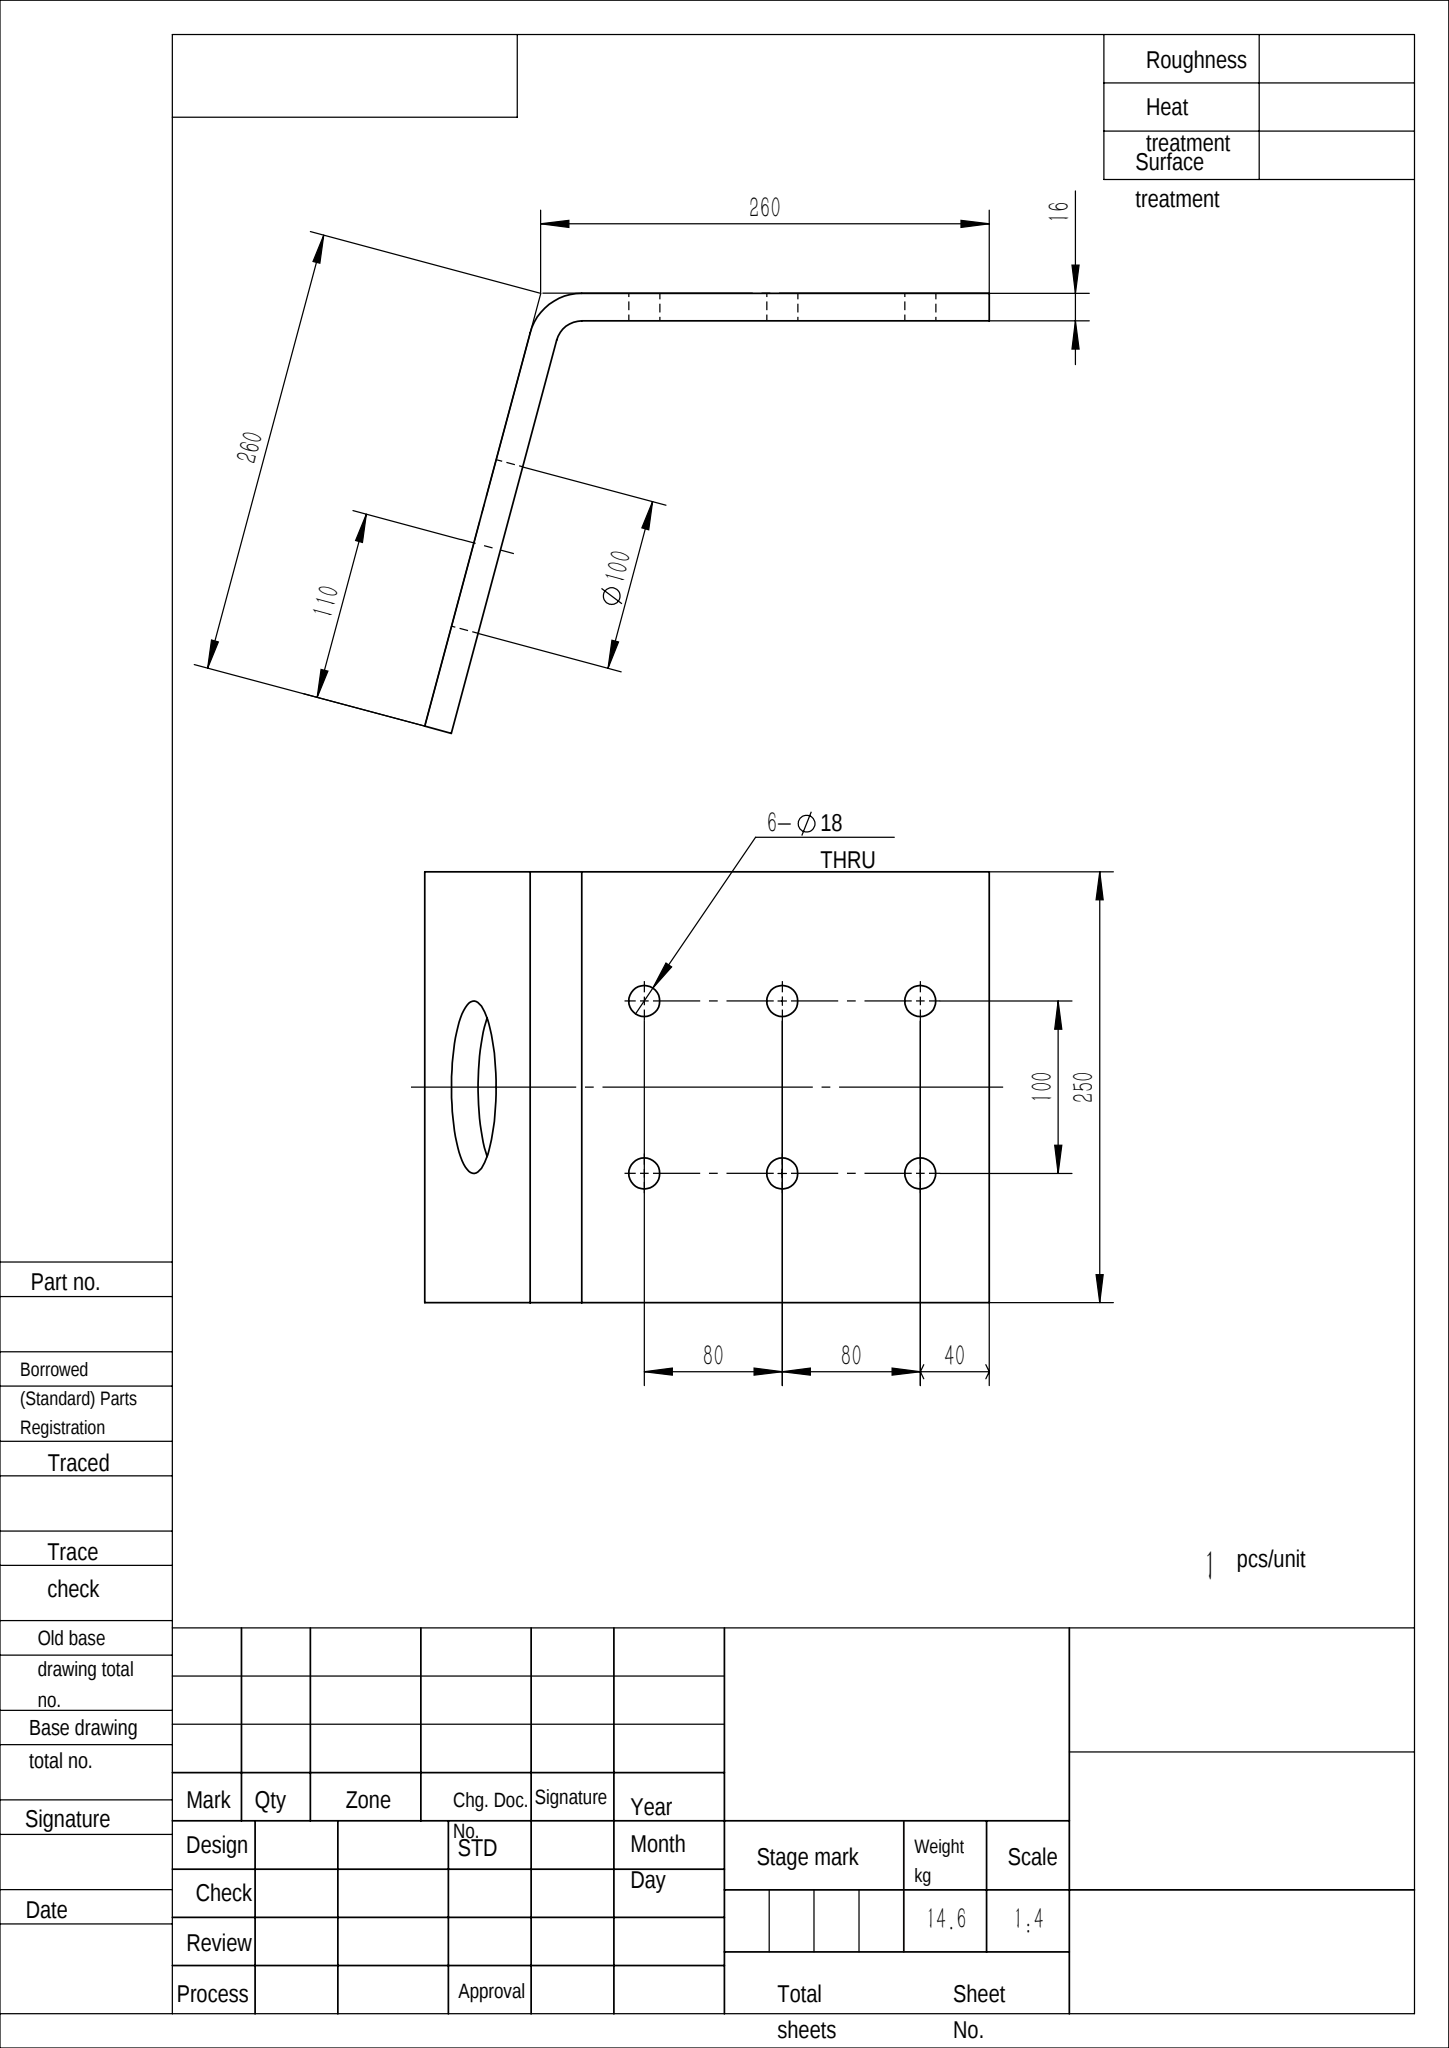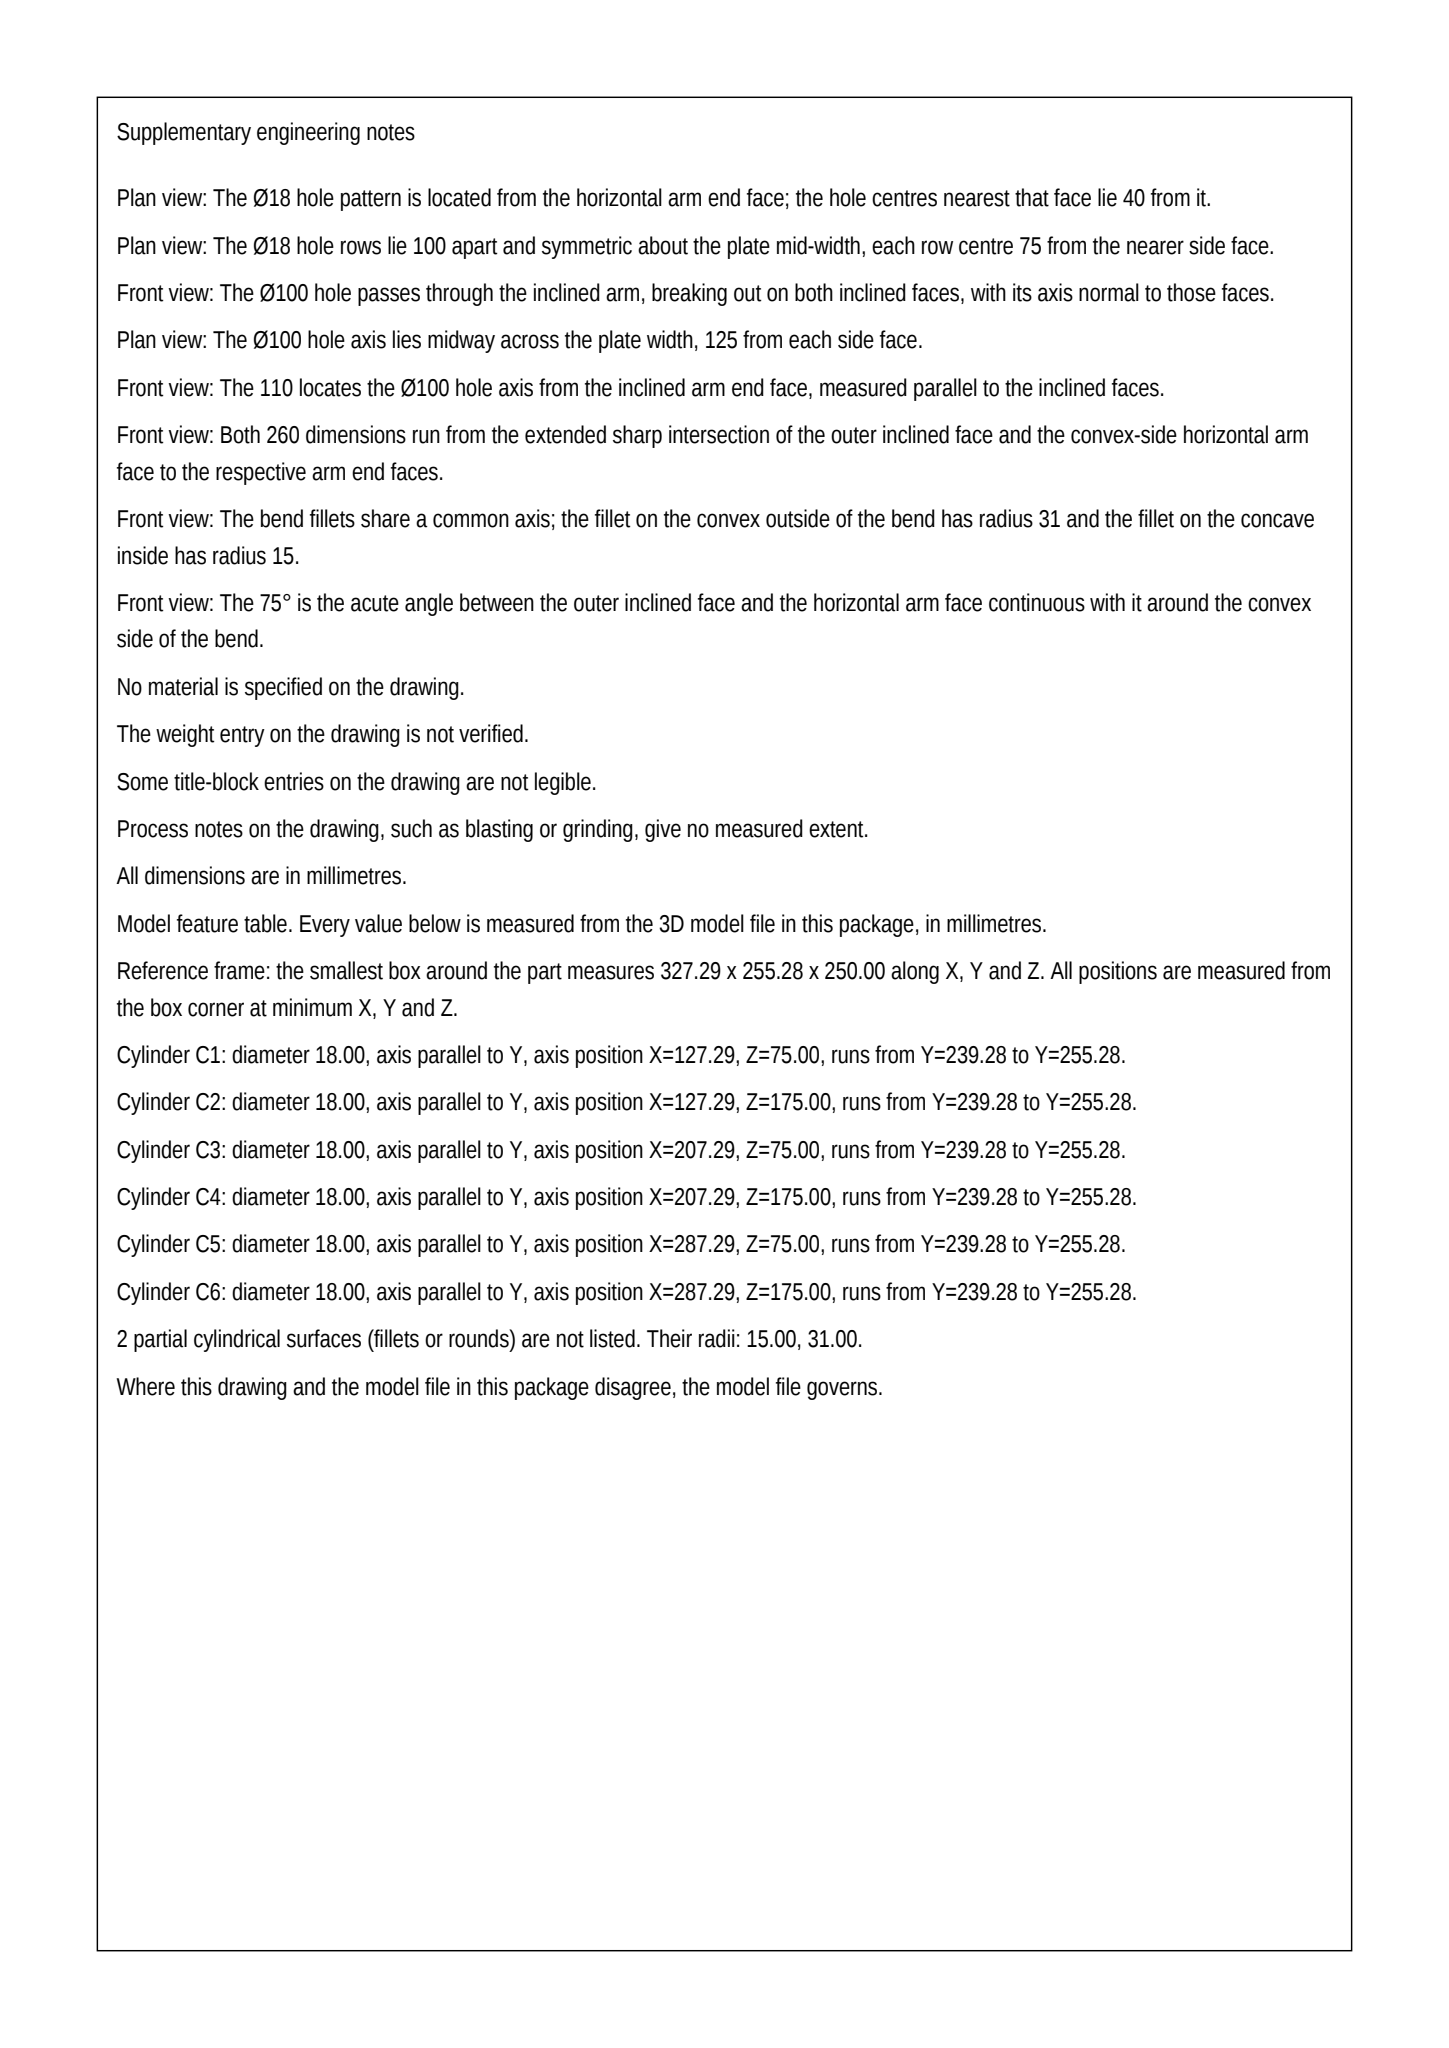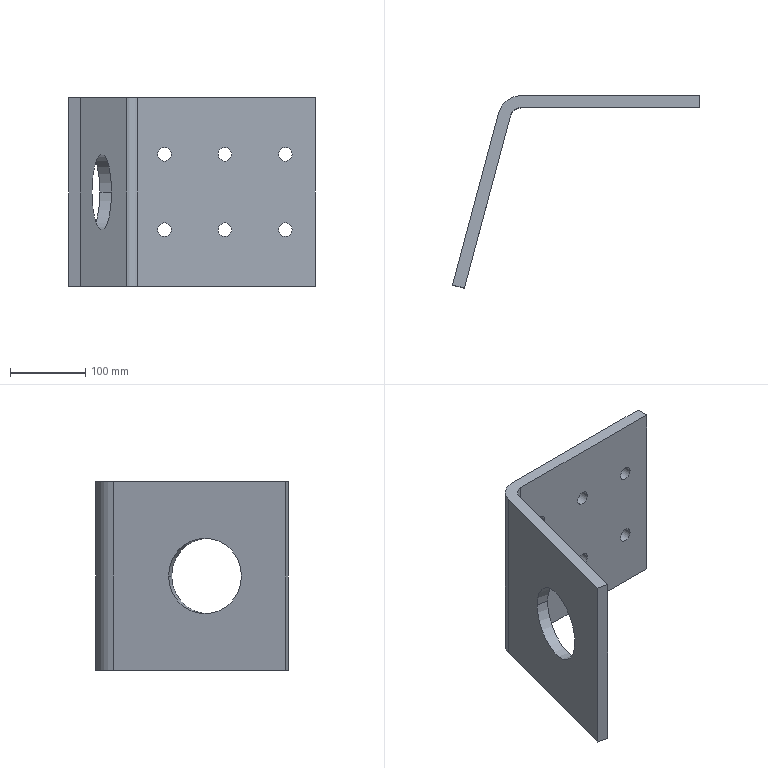Part | SolidWorks | mm | 1 solid | 24 faces | box 327.29 x 255.28 x 250 mm | volume 1860038 mm3 | cylinder 16 | plane 8 | commonest cylinder face diameters 18 x12 100 x2 30 x1 62 x1
Drawing notes:
INCLINED ARM THK 16 (UNIFORM W/ HORIZ ARM) | from the solid: Parallel faces y=239.28 & y=255.28 give 16 wall; holes len 16
① BEND ANGLE 105° BETWEEN FLAT ARM & INCLINED ARM | from the solid: Bent plate, t=16 (y 239.28 to 255.28), 250 wide (z 0 to 250); inclined arm meets horizontal arm at 105° included angle per model geometry
② R15 INSIDE BEND RAD AT 105° BEND | from the solid: Bend transition on 16 thk plate; inner bend face radius 15 (outer = 31)
build123d program:
from build123d import *

# Parameters (mm, degrees)
BOSS_EXTRUDE1_DEPTH = 125
CUT_EXTRUDE1_REACH  = 387.219
SKETCH2_R           = 9
LPATTERN1_COUNT     = 3
LPATTERN1_PITCH     = 80
SKETCH3_R           = 50
CUT_EXTRUDE2_DEPTH  = 373.155


with BuildPart() as part:
    # Sketch1 → Boss-Extrude1 (new, symmetric)
    with BuildSketch(Plane.XY):
        with BuildLine():
            Line((-67.293, -251.141), (-6.157, -22.977))
            ThreePointArc((-6.157, -22.977), (4.916, -6.406), (23.787, 0))
            Line((23.787, 0), (260, 0))
            Line((260, 0), (260, -16))
            Line((260, -16), (23.787, -16))
            ThreePointArc((23.787, -16), (14.656, -19.1), (9.298, -27.118))
            Line((9.298, -27.118), (-51.838, -255.282))
            Line((-51.838, -255.282), (-67.293, -251.141))
        make_face()
    extrude(amount=BOSS_EXTRUDE1_DEPTH, both=True)

    # Sketch2 → Cut-Extrude1 (cut, up to next)
    with BuildSketch(Plane(origin=(0, 0, 0), x_dir=(1, 0, 0), z_dir=(0, 1, 0)), mode=Mode.PRIVATE) as cut_extrude1_sk1:
        with Locations(Location((220, 50, 0), (0, 0, 180))):
            Circle(SKETCH2_R)
    cut_extrude1_tool1 = extrude(cut_extrude1_sk1.sketch, amount=-CUT_EXTRUDE1_REACH, mode=Mode.PRIVATE) & part.part
    # Sketch2 → Cut-Extrude1 (cut, up to next)
    with BuildSketch(Plane(origin=(0, 0, 0), x_dir=(1, 0, 0), z_dir=(0, 1, 0)), mode=Mode.PRIVATE) as cut_extrude1_sk2:
        with Locations(Location((220, -50, 0), (0, 0, 180))):
            Circle(SKETCH2_R)
    cut_extrude1_tool2 = extrude(cut_extrude1_sk2.sketch, amount=-CUT_EXTRUDE1_REACH, mode=Mode.PRIVATE) & part.part
    cut_extrude1_1 = cut_extrude1_tool1.solids().sort_by_distance((220, 0, -50))[0]
    add(cut_extrude1_1, mode=Mode.SUBTRACT)
    cut_extrude1_2 = cut_extrude1_tool2.solids().sort_by_distance((220, 0, 50))[0]
    add(cut_extrude1_2, mode=Mode.SUBTRACT)
    cut_extrude1 = cut_extrude1_1 + cut_extrude1_2  # Cut-Extrude1 as one shape, for the pattern or mirror that repeats it

    # LPattern1: Cut-Extrude1 ×3
    with Locations(*[(-i * LPATTERN1_PITCH, 0, 0) for i in range(1, LPATTERN1_COUNT)]):
        add(cut_extrude1, mode=Mode.SUBTRACT)

    # Sketch3 → Cut-Extrude2 (cut, through all)
    with BuildSketch(Plane(origin=(15.455, -4.141, 0), x_dir=(0, 0, -1), z_dir=(0.9659, -0.2588, 0))):
        with Locations(Location((0, -150, 0), (0, 0, 90))):
            Circle(SKETCH3_R)
    extrude(amount=-CUT_EXTRUDE2_DEPTH, mode=Mode.SUBTRACT)


solid = part.part
STEP:
#1=CARTESIAN_POINT('',(-51.764,-193.185,0.));
#2=VERTEX_POINT('',#1);
#3=CARTESIAN_POINT('',(-25.882,-96.593,-0.));
#4=VERTEX_POINT('',#3);
#5=CARTESIAN_POINT('',(-38.823,-144.889,0.));
#6=DIRECTION('',(0.9659,-0.2588,-0.));
#7=DIRECTION('',(0.2588,0.9659,0.));
#8=AXIS2_PLACEMENT_3D('',#5,#6,#7);
#9=CIRCLE('',#8,50.);
#10=EDGE_CURVE('',#2,#4,#9,.T.);
#11=ORIENTED_EDGE('',*,*,#10,.F.);
#12=CARTESIAN_POINT('',(-36.309,-197.326,0.));
#13=VERTEX_POINT('',#12);
#14=CARTESIAN_POINT('',(-114.549,-176.362,0.));
#15=DIRECTION('',(0.9659,-0.2588,-0.));
#16=VECTOR('',#15,1000.);
#17=LINE('',#14,#16);
#18=EDGE_CURVE('',#2,#13,#17,.T.);
#19=ORIENTED_EDGE('',*,*,#18,.T.);
#20=CARTESIAN_POINT('',(-10.427,-100.734,-0.));
#21=VERTEX_POINT('',#20);
#22=CARTESIAN_POINT('',(-23.368,-149.03,-0.));
#23=DIRECTION('',(0.9659,-0.2588,-0.));
#24=DIRECTION('',(0.2588,0.9659,0.));
#25=AXIS2_PLACEMENT_3D('',#22,#23,#24);
#26=CIRCLE('',#25,50.);
#27=EDGE_CURVE('',#13,#21,#26,.T.);
#28=ORIENTED_EDGE('',*,*,#27,.T.);
#29=CARTESIAN_POINT('',(-88.667,-79.769,0.));
#30=DIRECTION('',(0.9659,-0.2588,-0.));
#31=VECTOR('',#30,1000.);
#32=LINE('',#29,#31);
#33=EDGE_CURVE('',#4,#21,#32,.T.);
#34=ORIENTED_EDGE('',*,*,#33,.F.);
#35=EDGE_LOOP('',(#11,#19,#28,#34));
#36=FACE_OUTER_BOUND('',#35,.T.);
#37=CARTESIAN_POINT('',(-101.608,-128.066,0.));
#38=DIRECTION('',(0.9659,-0.2588,-0.));
#39=DIRECTION('',(0.2588,0.9659,0.));
#40=AXIS2_PLACEMENT_3D('',#37,#38,#39);
#41=CYLINDRICAL_SURFACE('',#40,50.);
#42=ADVANCED_FACE('',(#36),#41,.F.);
#43=CARTESIAN_POINT('',(131.,-16.,-50.));
#44=VERTEX_POINT('',#43);
#45=CARTESIAN_POINT('',(149.,-16.,-50.));
#46=VERTEX_POINT('',#45);
#47=CARTESIAN_POINT('',(140.,-16.,-50.));
#48=DIRECTION('',(0.,-1.,-0.));
#49=DIRECTION('',(-1.,-0.,0.));
#50=AXIS2_PLACEMENT_3D('',#47,#48,#49);
#51=CIRCLE('',#50,9.);
#52=EDGE_CURVE('',#44,#46,#51,.T.);
#53=ORIENTED_EDGE('',*,*,#52,.T.);
#54=CARTESIAN_POINT('',(149.,-0.,-50.));
#55=VERTEX_POINT('',#54);
#56=CARTESIAN_POINT('',(149.,-255.283,-50.));
#57=DIRECTION('',(-0.,1.,0.));
#58=VECTOR('',#57,1000.);
#59=LINE('',#56,#58);
#60=EDGE_CURVE('',#46,#55,#59,.T.);
#61=ORIENTED_EDGE('',*,*,#60,.T.);
#62=CARTESIAN_POINT('',(131.,-0.,-50.));
#63=VERTEX_POINT('',#62);
#64=CARTESIAN_POINT('',(140.,-0.,-50.));
#65=DIRECTION('',(-0.,1.,0.));
#66=DIRECTION('',(-1.,-0.,0.));
#67=AXIS2_PLACEMENT_3D('',#64,#65,#66);
#68=CIRCLE('',#67,9.);
#69=EDGE_CURVE('',#55,#63,#68,.T.);
#70=ORIENTED_EDGE('',*,*,#69,.T.);
#71=CARTESIAN_POINT('',(131.,-255.283,-50.));
#72=DIRECTION('',(-0.,1.,0.));
#73=VECTOR('',#72,1000.);
#74=LINE('',#71,#73);
#75=EDGE_CURVE('',#44,#63,#74,.T.);
#76=ORIENTED_EDGE('',*,*,#75,.F.);
#77=EDGE_LOOP('',(#53,#61,#70,#76));
#78=FACE_OUTER_BOUND('',#77,.T.);
#79=CARTESIAN_POINT('',(140.,-255.283,-50.));
#80=DIRECTION('',(-0.,1.,0.));
#81=DIRECTION('',(-1.,0.,0.));
#82=AXIS2_PLACEMENT_3D('',#79,#80,#81);
#83=CYLINDRICAL_SURFACE('',#82,9.);
#84=ADVANCED_FACE('',(#78),#83,.F.);
#85=CARTESIAN_POINT('',(131.,-16.,50.));
#86=VERTEX_POINT('',#85);
#87=CARTESIAN_POINT('',(149.,-16.,50.));
#88=VERTEX_POINT('',#87);
#89=CARTESIAN_POINT('',(140.,-16.,50.));
#90=DIRECTION('',(0.,-1.,-0.));
#91=DIRECTION('',(-1.,-0.,0.));
#92=AXIS2_PLACEMENT_3D('',#89,#90,#91);
#93=CIRCLE('',#92,9.);
#94=EDGE_CURVE('',#86,#88,#93,.T.);
#95=ORIENTED_EDGE('',*,*,#94,.T.);
#96=CARTESIAN_POINT('',(149.,-0.,50.));
#97=VERTEX_POINT('',#96);
#98=CARTESIAN_POINT('',(149.,-255.283,50.));
#99=DIRECTION('',(-0.,1.,0.));
#100=VECTOR('',#99,1000.);
#101=LINE('',#98,#100);
#102=EDGE_CURVE('',#88,#97,#101,.T.);
#103=ORIENTED_EDGE('',*,*,#102,.T.);
#104=CARTESIAN_POINT('',(131.,-0.,50.));
#105=VERTEX_POINT('',#104);
#106=CARTESIAN_POINT('',(140.,-0.,50.));
#107=DIRECTION('',(-0.,1.,0.));
#108=DIRECTION('',(-1.,-0.,0.));
#109=AXIS2_PLACEMENT_3D('',#106,#107,#108);
#110=CIRCLE('',#109,9.);
#111=EDGE_CURVE('',#97,#105,#110,.T.);
#112=ORIENTED_EDGE('',*,*,#111,.T.);
#113=CARTESIAN_POINT('',(131.,-255.283,50.));
#114=DIRECTION('',(-0.,1.,0.));
#115=VECTOR('',#114,1000.);
#116=LINE('',#113,#115);
#117=EDGE_CURVE('',#86,#105,#116,.T.);
#118=ORIENTED_EDGE('',*,*,#117,.F.);
#119=EDGE_LOOP('',(#95,#103,#112,#118));
#120=FACE_OUTER_BOUND('',#119,.T.);
#121=CARTESIAN_POINT('',(140.,-255.283,50.));
#122=DIRECTION('',(-0.,1.,0.));
#123=DIRECTION('',(-1.,0.,0.));
#124=AXIS2_PLACEMENT_3D('',#121,#122,#123);
#125=CYLINDRICAL_SURFACE('',#124,9.);
#126=ADVANCED_FACE('',(#120),#125,.F.);
#127=CARTESIAN_POINT('',(211.,-16.,50.));
#128=VERTEX_POINT('',#127);
#129=CARTESIAN_POINT('',(229.,-16.,50.));
#130=VERTEX_POINT('',#129);
#131=CARTESIAN_POINT('',(220.,-16.,50.));
#132=DIRECTION('',(0.,-1.,-0.));
#133=DIRECTION('',(-1.,-0.,0.));
#134=AXIS2_PLACEMENT_3D('',#131,#132,#133);
#135=CIRCLE('',#134,9.);
#136=EDGE_CURVE('',#128,#130,#135,.T.);
#137=ORIENTED_EDGE('',*,*,#136,.T.);
#138=CARTESIAN_POINT('',(229.,0.,50.));
#139=VERTEX_POINT('',#138);
#140=CARTESIAN_POINT('',(229.,-255.283,50.));
#141=DIRECTION('',(-0.,1.,0.));
#142=VECTOR('',#141,1000.);
#143=LINE('',#140,#142);
#144=EDGE_CURVE('',#130,#139,#143,.T.);
#145=ORIENTED_EDGE('',*,*,#144,.T.);
#146=CARTESIAN_POINT('',(211.,-0.,50.));
#147=VERTEX_POINT('',#146);
#148=CARTESIAN_POINT('',(220.,0.,50.));
#149=DIRECTION('',(-0.,1.,0.));
#150=DIRECTION('',(-1.,-0.,0.));
#151=AXIS2_PLACEMENT_3D('',#148,#149,#150);
#152=CIRCLE('',#151,9.);
#153=EDGE_CURVE('',#139,#147,#152,.T.);
#154=ORIENTED_EDGE('',*,*,#153,.T.);
#155=CARTESIAN_POINT('',(211.,-255.283,50.));
#156=DIRECTION('',(-0.,1.,0.));
#157=VECTOR('',#156,1000.);
#158=LINE('',#155,#157);
#159=EDGE_CURVE('',#128,#147,#158,.T.);
#160=ORIENTED_EDGE('',*,*,#159,.F.);
#161=EDGE_LOOP('',(#137,#145,#154,#160));
#162=FACE_OUTER_BOUND('',#161,.T.);
#163=CARTESIAN_POINT('',(220.,-255.283,50.));
#164=DIRECTION('',(-0.,1.,0.));
#165=DIRECTION('',(-1.,0.,0.));
#166=AXIS2_PLACEMENT_3D('',#163,#164,#165);
#167=CYLINDRICAL_SURFACE('',#166,9.);
#168=ADVANCED_FACE('',(#162),#167,.F.);
#169=CARTESIAN_POINT('',(211.,-16.,-50.));
#170=VERTEX_POINT('',#169);
#171=CARTESIAN_POINT('',(229.,-16.,-50.));
#172=VERTEX_POINT('',#171);
#173=CARTESIAN_POINT('',(220.,-16.,-50.));
#174=DIRECTION('',(0.,-1.,-0.));
#175=DIRECTION('',(-1.,-0.,0.));
#176=AXIS2_PLACEMENT_3D('',#173,#174,#175);
#177=CIRCLE('',#176,9.);
#178=EDGE_CURVE('',#170,#172,#177,.T.);
#179=ORIENTED_EDGE('',*,*,#178,.T.);
#180=CARTESIAN_POINT('',(229.,0.,-50.));
#181=VERTEX_POINT('',#180);
#182=CARTESIAN_POINT('',(229.,-255.283,-50.));
#183=DIRECTION('',(-0.,1.,0.));
#184=VECTOR('',#183,1000.);
#185=LINE('',#182,#184);
#186=EDGE_CURVE('',#172,#181,#185,.T.);
#187=ORIENTED_EDGE('',*,*,#186,.T.);
#188=CARTESIAN_POINT('',(211.,-0.,-50.));
#189=VERTEX_POINT('',#188);
#190=CARTESIAN_POINT('',(220.,0.,-50.));
#191=DIRECTION('',(-0.,1.,0.));
#192=DIRECTION('',(-1.,-0.,0.));
#193=AXIS2_PLACEMENT_3D('',#190,#191,#192);
#194=CIRCLE('',#193,9.);
#195=EDGE_CURVE('',#181,#189,#194,.T.);
#196=ORIENTED_EDGE('',*,*,#195,.T.);
#197=CARTESIAN_POINT('',(211.,-255.283,-50.));
#198=DIRECTION('',(-0.,1.,0.));
#199=VECTOR('',#198,1000.);
#200=LINE('',#197,#199);
#201=EDGE_CURVE('',#170,#189,#200,.T.);
#202=ORIENTED_EDGE('',*,*,#201,.F.);
#203=EDGE_LOOP('',(#179,#187,#196,#202));
#204=FACE_OUTER_BOUND('',#203,.T.);
#205=CARTESIAN_POINT('',(220.,-255.283,-50.));
#206=DIRECTION('',(-0.,1.,0.));
#207=DIRECTION('',(-1.,0.,0.));
#208=AXIS2_PLACEMENT_3D('',#205,#206,#207);
#209=CYLINDRICAL_SURFACE('',#208,9.);
#210=ADVANCED_FACE('',(#204),#209,.F.);
#211=CARTESIAN_POINT('',(51.,-16.,50.));
#212=VERTEX_POINT('',#211);
#213=CARTESIAN_POINT('',(69.,-16.,50.));
#214=VERTEX_POINT('',#213);
#215=CARTESIAN_POINT('',(60.,-16.,50.));
#216=DIRECTION('',(0.,-1.,-0.));
#217=DIRECTION('',(-1.,-0.,0.));
#218=AXIS2_PLACEMENT_3D('',#215,#216,#217);
#219=CIRCLE('',#218,9.);
#220=EDGE_CURVE('',#212,#214,#219,.T.);
#221=ORIENTED_EDGE('',*,*,#220,.T.);
#222=CARTESIAN_POINT('',(69.,0.,50.));
#223=VERTEX_POINT('',#222);
#224=CARTESIAN_POINT('',(69.,-255.283,50.));
#225=DIRECTION('',(-0.,1.,0.));
#226=VECTOR('',#225,1000.);
#227=LINE('',#224,#226);
#228=EDGE_CURVE('',#214,#223,#227,.T.);
#229=ORIENTED_EDGE('',*,*,#228,.T.);
#230=CARTESIAN_POINT('',(51.,-0.,50.));
#231=VERTEX_POINT('',#230);
#232=CARTESIAN_POINT('',(60.,0.,50.));
#233=DIRECTION('',(-0.,1.,0.));
#234=DIRECTION('',(-1.,-0.,0.));
#235=AXIS2_PLACEMENT_3D('',#232,#233,#234);
#236=CIRCLE('',#235,9.);
#237=EDGE_CURVE('',#223,#231,#236,.T.);
#238=ORIENTED_EDGE('',*,*,#237,.T.);
#239=CARTESIAN_POINT('',(51.,-255.283,50.));
#240=DIRECTION('',(-0.,1.,0.));
#241=VECTOR('',#240,1000.);
#242=LINE('',#239,#241);
#243=EDGE_CURVE('',#212,#231,#242,.T.);
#244=ORIENTED_EDGE('',*,*,#243,.F.);
#245=EDGE_LOOP('',(#221,#229,#238,#244));
#246=FACE_OUTER_BOUND('',#245,.T.);
#247=CARTESIAN_POINT('',(60.,-255.283,50.));
#248=DIRECTION('',(-0.,1.,0.));
#249=DIRECTION('',(-1.,0.,0.));
#250=AXIS2_PLACEMENT_3D('',#247,#248,#249);
#251=CYLINDRICAL_SURFACE('',#250,9.);
#252=ADVANCED_FACE('',(#246),#251,.F.);
#253=CARTESIAN_POINT('',(51.,-16.,-50.));
#254=VERTEX_POINT('',#253);
#255=CARTESIAN_POINT('',(69.,-16.,-50.));
#256=VERTEX_POINT('',#255);
#257=CARTESIAN_POINT('',(60.,-16.,-50.));
#258=DIRECTION('',(0.,-1.,-0.));
#259=DIRECTION('',(-1.,-0.,0.));
#260=AXIS2_PLACEMENT_3D('',#257,#258,#259);
#261=CIRCLE('',#260,9.);
#262=EDGE_CURVE('',#254,#256,#261,.T.);
#263=ORIENTED_EDGE('',*,*,#262,.T.);
#264=CARTESIAN_POINT('',(69.,0.,-50.));
#265=VERTEX_POINT('',#264);
#266=CARTESIAN_POINT('',(69.,-255.283,-50.));
#267=DIRECTION('',(-0.,1.,0.));
#268=VECTOR('',#267,1000.);
#269=LINE('',#266,#268);
#270=EDGE_CURVE('',#256,#265,#269,.T.);
#271=ORIENTED_EDGE('',*,*,#270,.T.);
#272=CARTESIAN_POINT('',(51.,-0.,-50.));
#273=VERTEX_POINT('',#272);
#274=CARTESIAN_POINT('',(60.,0.,-50.));
#275=DIRECTION('',(-0.,1.,0.));
#276=DIRECTION('',(-1.,-0.,0.));
#277=AXIS2_PLACEMENT_3D('',#274,#275,#276);
#278=CIRCLE('',#277,9.);
#279=EDGE_CURVE('',#265,#273,#278,.T.);
#280=ORIENTED_EDGE('',*,*,#279,.T.);
#281=CARTESIAN_POINT('',(51.,-255.283,-50.));
#282=DIRECTION('',(-0.,1.,0.));
#283=VECTOR('',#282,1000.);
#284=LINE('',#281,#283);
#285=EDGE_CURVE('',#254,#273,#284,.T.);
#286=ORIENTED_EDGE('',*,*,#285,.F.);
#287=EDGE_LOOP('',(#263,#271,#280,#286));
#288=FACE_OUTER_BOUND('',#287,.T.);
#289=CARTESIAN_POINT('',(60.,-255.283,-50.));
#290=DIRECTION('',(-0.,1.,0.));
#291=DIRECTION('',(-1.,0.,0.));
#292=AXIS2_PLACEMENT_3D('',#289,#290,#291);
#293=CYLINDRICAL_SURFACE('',#292,9.);
#294=ADVANCED_FACE('',(#288),#293,.F.);
#295=ORIENTED_EDGE('',*,*,#270,.F.);
#296=CARTESIAN_POINT('',(60.,-16.,-50.));
#297=DIRECTION('',(0.,-1.,-0.));
#298=DIRECTION('',(-1.,-0.,0.));
#299=AXIS2_PLACEMENT_3D('',#296,#297,#298);
#300=CIRCLE('',#299,9.);
#301=EDGE_CURVE('',#256,#254,#300,.T.);
#302=ORIENTED_EDGE('',*,*,#301,.T.);
#303=ORIENTED_EDGE('',*,*,#285,.T.);
#304=CARTESIAN_POINT('',(60.,0.,-50.));
#305=DIRECTION('',(-0.,1.,0.));
#306=DIRECTION('',(-1.,-0.,0.));
#307=AXIS2_PLACEMENT_3D('',#304,#305,#306);
#308=CIRCLE('',#307,9.);
#309=EDGE_CURVE('',#273,#265,#308,.T.);
#310=ORIENTED_EDGE('',*,*,#309,.T.);
#311=EDGE_LOOP('',(#295,#302,#303,#310));
#312=FACE_OUTER_BOUND('',#311,.T.);
#313=CARTESIAN_POINT('',(60.,-255.283,-50.));
#314=DIRECTION('',(-0.,1.,0.));
#315=DIRECTION('',(-1.,0.,0.));
#316=AXIS2_PLACEMENT_3D('',#313,#314,#315);
#317=CYLINDRICAL_SURFACE('',#316,9.);
#318=ADVANCED_FACE('',(#312),#317,.F.);
#319=ORIENTED_EDGE('',*,*,#228,.F.);
#320=CARTESIAN_POINT('',(60.,-16.,50.));
#321=DIRECTION('',(0.,-1.,-0.));
#322=DIRECTION('',(-1.,-0.,0.));
#323=AXIS2_PLACEMENT_3D('',#320,#321,#322);
#324=CIRCLE('',#323,9.);
#325=EDGE_CURVE('',#214,#212,#324,.T.);
#326=ORIENTED_EDGE('',*,*,#325,.T.);
#327=ORIENTED_EDGE('',*,*,#243,.T.);
#328=CARTESIAN_POINT('',(60.,0.,50.));
#329=DIRECTION('',(-0.,1.,0.));
#330=DIRECTION('',(-1.,-0.,0.));
#331=AXIS2_PLACEMENT_3D('',#328,#329,#330);
#332=CIRCLE('',#331,9.);
#333=EDGE_CURVE('',#231,#223,#332,.T.);
#334=ORIENTED_EDGE('',*,*,#333,.T.);
#335=EDGE_LOOP('',(#319,#326,#327,#334));
#336=FACE_OUTER_BOUND('',#335,.T.);
#337=CARTESIAN_POINT('',(60.,-255.283,50.));
#338=DIRECTION('',(-0.,1.,0.));
#339=DIRECTION('',(-1.,0.,0.));
#340=AXIS2_PLACEMENT_3D('',#337,#338,#339);
#341=CYLINDRICAL_SURFACE('',#340,9.);
#342=ADVANCED_FACE('',(#336),#341,.F.);
#343=CARTESIAN_POINT('',(-67.293,-251.141,-125.));
#344=VERTEX_POINT('',#343);
#345=CARTESIAN_POINT('',(-51.838,-255.282,-125.));
#346=VERTEX_POINT('',#345);
#347=CARTESIAN_POINT('',(-51.838,-255.282,-125.));
#348=DIRECTION('',(0.9659,-0.2588,-0.));
#349=VECTOR('',#348,1000.);
#350=LINE('',#347,#349);
#351=EDGE_CURVE('',#344,#346,#350,.T.);
#352=ORIENTED_EDGE('',*,*,#351,.T.);
#353=CARTESIAN_POINT('',(-51.838,-255.282,125.));
#354=VERTEX_POINT('',#353);
#355=CARTESIAN_POINT('',(-51.838,-255.282,125.));
#356=DIRECTION('',(0.,-0.,-1.));
#357=VECTOR('',#356,1000.);
#358=LINE('',#355,#357);
#359=EDGE_CURVE('',#354,#346,#358,.T.);
#360=ORIENTED_EDGE('',*,*,#359,.F.);
#361=CARTESIAN_POINT('',(-67.293,-251.141,125.));
#362=VERTEX_POINT('',#361);
#363=CARTESIAN_POINT('',(-51.838,-255.282,125.));
#364=DIRECTION('',(0.9659,-0.2588,-0.));
#365=VECTOR('',#364,1000.);
#366=LINE('',#363,#365);
#367=EDGE_CURVE('',#362,#354,#366,.T.);
#368=ORIENTED_EDGE('',*,*,#367,.F.);
#369=CARTESIAN_POINT('',(-67.293,-251.141,125.));
#370=DIRECTION('',(0.,-0.,-1.));
#371=VECTOR('',#370,1000.);
#372=LINE('',#369,#371);
#373=EDGE_CURVE('',#362,#344,#372,.T.);
#374=ORIENTED_EDGE('',*,*,#373,.T.);
#375=EDGE_LOOP('',(#352,#360,#368,#374));
#376=FACE_OUTER_BOUND('',#375,.T.);
#377=CARTESIAN_POINT('',(-51.838,-255.282,125.));
#378=DIRECTION('',(0.2588,0.9659,0.));
#379=DIRECTION('',(-0.9659,0.2588,0.));
#380=AXIS2_PLACEMENT_3D('',#377,#378,#379);
#381=PLANE('',#380);
#382=ADVANCED_FACE('',(#376),#381,.F.);
#383=CARTESIAN_POINT('',(-23.368,-149.03,-0.));
#384=DIRECTION('',(0.9659,-0.2588,-0.));
#385=DIRECTION('',(0.2588,0.9659,0.));
#386=AXIS2_PLACEMENT_3D('',#383,#384,#385);
#387=CIRCLE('',#386,50.);
#388=EDGE_CURVE('',#21,#13,#387,.T.);
#389=ORIENTED_EDGE('',*,*,#388,.F.);
#390=ORIENTED_EDGE('',*,*,#27,.F.);
#391=EDGE_LOOP('',(#389,#390));
#392=FACE_BOUND('',#391,.T.);
#393=CARTESIAN_POINT('',(9.298,-27.118,-125.));
#394=VERTEX_POINT('',#393);
#395=CARTESIAN_POINT('',(9.298,-27.118,-125.));
#396=DIRECTION('',(0.2588,0.9659,0.));
#397=VECTOR('',#396,1000.);
#398=LINE('',#395,#397);
#399=EDGE_CURVE('',#346,#394,#398,.T.);
#400=ORIENTED_EDGE('',*,*,#399,.T.);
#401=CARTESIAN_POINT('',(9.298,-27.118,125.));
#402=VERTEX_POINT('',#401);
#403=CARTESIAN_POINT('',(9.298,-27.118,125.));
#404=DIRECTION('',(0.,-0.,-1.));
#405=VECTOR('',#404,1000.);
#406=LINE('',#403,#405);
#407=EDGE_CURVE('',#402,#394,#406,.T.);
#408=ORIENTED_EDGE('',*,*,#407,.F.);
#409=CARTESIAN_POINT('',(9.298,-27.118,125.));
#410=DIRECTION('',(0.2588,0.9659,0.));
#411=VECTOR('',#410,1000.);
#412=LINE('',#409,#411);
#413=EDGE_CURVE('',#354,#402,#412,.T.);
#414=ORIENTED_EDGE('',*,*,#413,.F.);
#415=ORIENTED_EDGE('',*,*,#359,.T.);
#416=EDGE_LOOP('',(#400,#408,#414,#415));
#417=FACE_OUTER_BOUND('',#416,.T.);
#418=CARTESIAN_POINT('',(9.298,-27.118,125.));
#419=DIRECTION('',(-0.9659,0.2588,0.));
#420=DIRECTION('',(-0.2588,-0.9659,0.));
#421=AXIS2_PLACEMENT_3D('',#418,#419,#420);
#422=PLANE('',#421);
#423=ADVANCED_FACE('',(#392,#417),#422,.F.);
#424=CARTESIAN_POINT('',(23.787,-16.,-125.));
#425=VERTEX_POINT('',#424);
#426=CARTESIAN_POINT('',(23.787,-31.,-125.));
#427=DIRECTION('',(0.,-0.,-1.));
#428=DIRECTION('',(-1.,0.,0.));
#429=AXIS2_PLACEMENT_3D('',#426,#427,#428);
#430=CIRCLE('',#429,15.);
#431=EDGE_CURVE('',#394,#425,#430,.T.);
#432=ORIENTED_EDGE('',*,*,#431,.T.);
#433=CARTESIAN_POINT('',(23.787,-16.,125.));
#434=VERTEX_POINT('',#433);
#435=CARTESIAN_POINT('',(23.787,-16.,125.));
#436=DIRECTION('',(0.,-0.,-1.));
#437=VECTOR('',#436,1000.);
#438=LINE('',#435,#437);
#439=EDGE_CURVE('',#434,#425,#438,.T.);
#440=ORIENTED_EDGE('',*,*,#439,.F.);
#441=CARTESIAN_POINT('',(23.787,-31.,125.));
#442=DIRECTION('',(0.,-0.,-1.));
#443=DIRECTION('',(-1.,0.,0.));
#444=AXIS2_PLACEMENT_3D('',#441,#442,#443);
#445=CIRCLE('',#444,15.);
#446=EDGE_CURVE('',#402,#434,#445,.T.);
#447=ORIENTED_EDGE('',*,*,#446,.F.);
#448=ORIENTED_EDGE('',*,*,#407,.T.);
#449=EDGE_LOOP('',(#432,#440,#447,#448));
#450=FACE_OUTER_BOUND('',#449,.T.);
#451=CARTESIAN_POINT('',(23.787,-31.,125.));
#452=DIRECTION('',(0.,-0.,-1.));
#453=DIRECTION('',(-1.,0.,0.));
#454=AXIS2_PLACEMENT_3D('',#451,#452,#453);
#455=CYLINDRICAL_SURFACE('',#454,15.);
#456=ADVANCED_FACE('',(#450),#455,.F.);
#457=ORIENTED_EDGE('',*,*,#52,.F.);
#458=CARTESIAN_POINT('',(140.,-16.,-50.));
#459=DIRECTION('',(0.,-1.,-0.));
#460=DIRECTION('',(-1.,-0.,0.));
#461=AXIS2_PLACEMENT_3D('',#458,#459,#460);
#462=CIRCLE('',#461,9.);
#463=EDGE_CURVE('',#46,#44,#462,.T.);
#464=ORIENTED_EDGE('',*,*,#463,.F.);
#465=EDGE_LOOP('',(#457,#464));
#466=FACE_BOUND('',#465,.T.);
#467=ORIENTED_EDGE('',*,*,#94,.F.);
#468=CARTESIAN_POINT('',(140.,-16.,50.));
#469=DIRECTION('',(0.,-1.,-0.));
#470=DIRECTION('',(-1.,-0.,0.));
#471=AXIS2_PLACEMENT_3D('',#468,#469,#470);
#472=CIRCLE('',#471,9.);
#473=EDGE_CURVE('',#88,#86,#472,.T.);
#474=ORIENTED_EDGE('',*,*,#473,.F.);
#475=EDGE_LOOP('',(#467,#474));
#476=FACE_BOUND('',#475,.T.);
#477=ORIENTED_EDGE('',*,*,#136,.F.);
#478=CARTESIAN_POINT('',(220.,-16.,50.));
#479=DIRECTION('',(0.,-1.,-0.));
#480=DIRECTION('',(-1.,-0.,0.));
#481=AXIS2_PLACEMENT_3D('',#478,#479,#480);
#482=CIRCLE('',#481,9.);
#483=EDGE_CURVE('',#130,#128,#482,.T.);
#484=ORIENTED_EDGE('',*,*,#483,.F.);
#485=EDGE_LOOP('',(#477,#484));
#486=FACE_BOUND('',#485,.T.);
#487=ORIENTED_EDGE('',*,*,#178,.F.);
#488=CARTESIAN_POINT('',(220.,-16.,-50.));
#489=DIRECTION('',(0.,-1.,-0.));
#490=DIRECTION('',(-1.,-0.,0.));
#491=AXIS2_PLACEMENT_3D('',#488,#489,#490);
#492=CIRCLE('',#491,9.);
#493=EDGE_CURVE('',#172,#170,#492,.T.);
#494=ORIENTED_EDGE('',*,*,#493,.F.);
#495=EDGE_LOOP('',(#487,#494));
#496=FACE_BOUND('',#495,.T.);
#497=CARTESIAN_POINT('',(260.,-16.,-125.));
#498=VERTEX_POINT('',#497);
#499=CARTESIAN_POINT('',(260.,-16.,-125.));
#500=DIRECTION('',(1.,0.,-0.));
#501=VECTOR('',#500,1000.);
#502=LINE('',#499,#501);
#503=EDGE_CURVE('',#425,#498,#502,.T.);
#504=ORIENTED_EDGE('',*,*,#503,.T.);
#505=CARTESIAN_POINT('',(260.,-16.,125.));
#506=VERTEX_POINT('',#505);
#507=CARTESIAN_POINT('',(260.,-16.,125.));
#508=DIRECTION('',(0.,-0.,-1.));
#509=VECTOR('',#508,1000.);
#510=LINE('',#507,#509);
#511=EDGE_CURVE('',#506,#498,#510,.T.);
#512=ORIENTED_EDGE('',*,*,#511,.F.);
#513=CARTESIAN_POINT('',(260.,-16.,125.));
#514=DIRECTION('',(1.,0.,-0.));
#515=VECTOR('',#514,1000.);
#516=LINE('',#513,#515);
#517=EDGE_CURVE('',#434,#506,#516,.T.);
#518=ORIENTED_EDGE('',*,*,#517,.F.);
#519=ORIENTED_EDGE('',*,*,#439,.T.);
#520=EDGE_LOOP('',(#504,#512,#518,#519));
#521=FACE_OUTER_BOUND('',#520,.T.);
#522=ORIENTED_EDGE('',*,*,#220,.F.);
#523=ORIENTED_EDGE('',*,*,#325,.F.);
#524=EDGE_LOOP('',(#522,#523));
#525=FACE_BOUND('',#524,.T.);
#526=ORIENTED_EDGE('',*,*,#262,.F.);
#527=ORIENTED_EDGE('',*,*,#301,.F.);
#528=EDGE_LOOP('',(#526,#527));
#529=FACE_BOUND('',#528,.T.);
#530=CARTESIAN_POINT('',(260.,-16.,125.));
#531=DIRECTION('',(-0.,1.,0.));
#532=DIRECTION('',(-1.,-0.,0.));
#533=AXIS2_PLACEMENT_3D('',#530,#531,#532);
#534=PLANE('',#533);
#535=ADVANCED_FACE('',(#466,#476,#486,#496,#521,#525,#529),#534,.F.);
#536=CARTESIAN_POINT('',(260.,-0.,-125.));
#537=VERTEX_POINT('',#536);
#538=CARTESIAN_POINT('',(260.,-0.,-125.));
#539=DIRECTION('',(0.,1.,0.));
#540=VECTOR('',#539,1000.);
#541=LINE('',#538,#540);
#542=EDGE_CURVE('',#498,#537,#541,.T.);
#543=ORIENTED_EDGE('',*,*,#542,.T.);
#544=CARTESIAN_POINT('',(260.,-0.,125.));
#545=VERTEX_POINT('',#544);
#546=CARTESIAN_POINT('',(260.,-0.,125.));
#547=DIRECTION('',(0.,-0.,-1.));
#548=VECTOR('',#547,1000.);
#549=LINE('',#546,#548);
#550=EDGE_CURVE('',#545,#537,#549,.T.);
#551=ORIENTED_EDGE('',*,*,#550,.F.);
#552=CARTESIAN_POINT('',(260.,-0.,125.));
#553=DIRECTION('',(0.,1.,0.));
#554=VECTOR('',#553,1000.);
#555=LINE('',#552,#554);
#556=EDGE_CURVE('',#506,#545,#555,.T.);
#557=ORIENTED_EDGE('',*,*,#556,.F.);
#558=ORIENTED_EDGE('',*,*,#511,.T.);
#559=EDGE_LOOP('',(#543,#551,#557,#558));
#560=FACE_OUTER_BOUND('',#559,.T.);
#561=CARTESIAN_POINT('',(260.,-0.,125.));
#562=DIRECTION('',(-1.,-0.,-0.));
#563=DIRECTION('',(-0.,0.,1.));
#564=AXIS2_PLACEMENT_3D('',#561,#562,#563);
#565=PLANE('',#564);
#566=ADVANCED_FACE('',(#560),#565,.F.);
#567=CARTESIAN_POINT('',(140.,-0.,-50.));
#568=DIRECTION('',(-0.,1.,0.));
#569=DIRECTION('',(-1.,-0.,0.));
#570=AXIS2_PLACEMENT_3D('',#567,#568,#569);
#571=CIRCLE('',#570,9.);
#572=EDGE_CURVE('',#63,#55,#571,.T.);
#573=ORIENTED_EDGE('',*,*,#572,.F.);
#574=ORIENTED_EDGE('',*,*,#69,.F.);
#575=EDGE_LOOP('',(#573,#574));
#576=FACE_BOUND('',#575,.T.);
#577=CARTESIAN_POINT('',(140.,-0.,50.));
#578=DIRECTION('',(-0.,1.,0.));
#579=DIRECTION('',(-1.,-0.,0.));
#580=AXIS2_PLACEMENT_3D('',#577,#578,#579);
#581=CIRCLE('',#580,9.);
#582=EDGE_CURVE('',#105,#97,#581,.T.);
#583=ORIENTED_EDGE('',*,*,#582,.F.);
#584=ORIENTED_EDGE('',*,*,#111,.F.);
#585=EDGE_LOOP('',(#583,#584));
#586=FACE_BOUND('',#585,.T.);
#587=CARTESIAN_POINT('',(220.,0.,50.));
#588=DIRECTION('',(-0.,1.,0.));
#589=DIRECTION('',(-1.,-0.,0.));
#590=AXIS2_PLACEMENT_3D('',#587,#588,#589);
#591=CIRCLE('',#590,9.);
#592=EDGE_CURVE('',#147,#139,#591,.T.);
#593=ORIENTED_EDGE('',*,*,#592,.F.);
#594=ORIENTED_EDGE('',*,*,#153,.F.);
#595=EDGE_LOOP('',(#593,#594));
#596=FACE_BOUND('',#595,.T.);
#597=CARTESIAN_POINT('',(220.,0.,-50.));
#598=DIRECTION('',(-0.,1.,0.));
#599=DIRECTION('',(-1.,-0.,0.));
#600=AXIS2_PLACEMENT_3D('',#597,#598,#599);
#601=CIRCLE('',#600,9.);
#602=EDGE_CURVE('',#189,#181,#601,.T.);
#603=ORIENTED_EDGE('',*,*,#602,.F.);
#604=ORIENTED_EDGE('',*,*,#195,.F.);
#605=EDGE_LOOP('',(#603,#604));
#606=FACE_BOUND('',#605,.T.);
#607=CARTESIAN_POINT('',(23.787,-0.,-125.));
#608=VERTEX_POINT('',#607);
#609=CARTESIAN_POINT('',(23.787,-0.,-125.));
#610=DIRECTION('',(-1.,-0.,0.));
#611=VECTOR('',#610,1000.);
#612=LINE('',#609,#611);
#613=EDGE_CURVE('',#537,#608,#612,.T.);
#614=ORIENTED_EDGE('',*,*,#613,.T.);
#615=CARTESIAN_POINT('',(23.787,-0.,125.));
#616=VERTEX_POINT('',#615);
#617=CARTESIAN_POINT('',(23.787,-0.,125.));
#618=DIRECTION('',(0.,-0.,-1.));
#619=VECTOR('',#618,1000.);
#620=LINE('',#617,#619);
#621=EDGE_CURVE('',#616,#608,#620,.T.);
#622=ORIENTED_EDGE('',*,*,#621,.F.);
#623=CARTESIAN_POINT('',(23.787,-0.,125.));
#624=DIRECTION('',(-1.,-0.,0.));
#625=VECTOR('',#624,1000.);
#626=LINE('',#623,#625);
#627=EDGE_CURVE('',#545,#616,#626,.T.);
#628=ORIENTED_EDGE('',*,*,#627,.F.);
#629=ORIENTED_EDGE('',*,*,#550,.T.);
#630=EDGE_LOOP('',(#614,#622,#628,#629));
#631=FACE_OUTER_BOUND('',#630,.T.);
#632=ORIENTED_EDGE('',*,*,#333,.F.);
#633=ORIENTED_EDGE('',*,*,#237,.F.);
#634=EDGE_LOOP('',(#632,#633));
#635=FACE_BOUND('',#634,.T.);
#636=ORIENTED_EDGE('',*,*,#309,.F.);
#637=ORIENTED_EDGE('',*,*,#279,.F.);
#638=EDGE_LOOP('',(#636,#637));
#639=FACE_BOUND('',#638,.T.);
#640=CARTESIAN_POINT('',(23.787,-0.,125.));
#641=DIRECTION('',(0.,-1.,-0.));
#642=DIRECTION('',(1.,0.,-0.));
#643=AXIS2_PLACEMENT_3D('',#640,#641,#642);
#644=PLANE('',#643);
#645=ADVANCED_FACE('',(#576,#586,#596,#606,#631,#635,#639),#644,.F.);
#646=CARTESIAN_POINT('',(-6.157,-22.977,-125.));
#647=VERTEX_POINT('',#646);
#648=CARTESIAN_POINT('',(23.787,-31.,-125.));
#649=DIRECTION('',(-0.,0.,1.));
#650=DIRECTION('',(-1.,0.,0.));
#651=AXIS2_PLACEMENT_3D('',#648,#649,#650);
#652=CIRCLE('',#651,31.);
#653=EDGE_CURVE('',#608,#647,#652,.T.);
#654=ORIENTED_EDGE('',*,*,#653,.T.);
#655=CARTESIAN_POINT('',(-6.157,-22.977,125.));
#656=VERTEX_POINT('',#655);
#657=CARTESIAN_POINT('',(-6.157,-22.977,125.));
#658=DIRECTION('',(0.,-0.,-1.));
#659=VECTOR('',#658,1000.);
#660=LINE('',#657,#659);
#661=EDGE_CURVE('',#656,#647,#660,.T.);
#662=ORIENTED_EDGE('',*,*,#661,.F.);
#663=CARTESIAN_POINT('',(23.787,-31.,125.));
#664=DIRECTION('',(-0.,0.,1.));
#665=DIRECTION('',(-1.,0.,0.));
#666=AXIS2_PLACEMENT_3D('',#663,#664,#665);
#667=CIRCLE('',#666,31.);
#668=EDGE_CURVE('',#616,#656,#667,.T.);
#669=ORIENTED_EDGE('',*,*,#668,.F.);
#670=ORIENTED_EDGE('',*,*,#621,.T.);
#671=EDGE_LOOP('',(#654,#662,#669,#670));
#672=FACE_OUTER_BOUND('',#671,.T.);
#673=CARTESIAN_POINT('',(23.787,-31.,125.));
#674=DIRECTION('',(0.,-0.,-1.));
#675=DIRECTION('',(-1.,0.,0.));
#676=AXIS2_PLACEMENT_3D('',#673,#674,#675);
#677=CYLINDRICAL_SURFACE('',#676,31.);
#678=ADVANCED_FACE('',(#672),#677,.T.);
#679=CARTESIAN_POINT('',(-38.823,-144.889,0.));
#680=DIRECTION('',(0.9659,-0.2588,-0.));
#681=DIRECTION('',(0.2588,0.9659,0.));
#682=AXIS2_PLACEMENT_3D('',#679,#680,#681);
#683=CIRCLE('',#682,50.);
#684=EDGE_CURVE('',#4,#2,#683,.T.);
#685=ORIENTED_EDGE('',*,*,#684,.T.);
#686=ORIENTED_EDGE('',*,*,#10,.T.);
#687=EDGE_LOOP('',(#685,#686));
#688=FACE_BOUND('',#687,.T.);
#689=CARTESIAN_POINT('',(-67.293,-251.141,-125.));
#690=DIRECTION('',(-0.2588,-0.9659,-0.));
#691=VECTOR('',#690,1000.);
#692=LINE('',#689,#691);
#693=EDGE_CURVE('',#647,#344,#692,.T.);
#694=ORIENTED_EDGE('',*,*,#693,.T.);
#695=ORIENTED_EDGE('',*,*,#373,.F.);
#696=CARTESIAN_POINT('',(-67.293,-251.141,125.));
#697=DIRECTION('',(-0.2588,-0.9659,-0.));
#698=VECTOR('',#697,1000.);
#699=LINE('',#696,#698);
#700=EDGE_CURVE('',#656,#362,#699,.T.);
#701=ORIENTED_EDGE('',*,*,#700,.F.);
#702=ORIENTED_EDGE('',*,*,#661,.T.);
#703=EDGE_LOOP('',(#694,#695,#701,#702));
#704=FACE_OUTER_BOUND('',#703,.T.);
#705=CARTESIAN_POINT('',(-67.293,-251.141,125.));
#706=DIRECTION('',(0.9659,-0.2588,-0.));
#707=DIRECTION('',(0.2588,0.9659,0.));
#708=AXIS2_PLACEMENT_3D('',#705,#706,#707);
#709=PLANE('',#708);
#710=ADVANCED_FACE('',(#688,#704),#709,.F.);
#711=ORIENTED_EDGE('',*,*,#367,.T.);
#712=ORIENTED_EDGE('',*,*,#413,.T.);
#713=ORIENTED_EDGE('',*,*,#446,.T.);
#714=ORIENTED_EDGE('',*,*,#517,.T.);
#715=ORIENTED_EDGE('',*,*,#556,.T.);
#716=ORIENTED_EDGE('',*,*,#627,.T.);
#717=ORIENTED_EDGE('',*,*,#668,.T.);
#718=ORIENTED_EDGE('',*,*,#700,.T.);
#719=EDGE_LOOP('',(#711,#712,#713,#714,#715,#716,#717,#718));
#720=FACE_OUTER_BOUND('',#719,.T.);
#721=CARTESIAN_POINT('',(23.787,-31.,125.));
#722=DIRECTION('',(-0.,-0.,-1.));
#723=DIRECTION('',(-1.,-0.,0.));
#724=AXIS2_PLACEMENT_3D('',#721,#722,#723);
#725=PLANE('',#724);
#726=ADVANCED_FACE('',(#720),#725,.F.);
#727=ORIENTED_EDGE('',*,*,#351,.F.);
#728=ORIENTED_EDGE('',*,*,#693,.F.);
#729=ORIENTED_EDGE('',*,*,#653,.F.);
#730=ORIENTED_EDGE('',*,*,#613,.F.);
#731=ORIENTED_EDGE('',*,*,#542,.F.);
#732=ORIENTED_EDGE('',*,*,#503,.F.);
#733=ORIENTED_EDGE('',*,*,#431,.F.);
#734=ORIENTED_EDGE('',*,*,#399,.F.);
#735=EDGE_LOOP('',(#727,#728,#729,#730,#731,#732,#733,#734));
#736=FACE_OUTER_BOUND('',#735,.T.);
#737=CARTESIAN_POINT('',(23.787,-31.,-125.));
#738=DIRECTION('',(-0.,-0.,-1.));
#739=DIRECTION('',(-1.,-0.,0.));
#740=AXIS2_PLACEMENT_3D('',#737,#738,#739);
#741=PLANE('',#740);
#742=ADVANCED_FACE('',(#736),#741,.T.);
#743=ORIENTED_EDGE('',*,*,#186,.F.);
#744=ORIENTED_EDGE('',*,*,#493,.T.);
#745=ORIENTED_EDGE('',*,*,#201,.T.);
#746=ORIENTED_EDGE('',*,*,#602,.T.);
#747=EDGE_LOOP('',(#743,#744,#745,#746));
#748=FACE_OUTER_BOUND('',#747,.T.);
#749=CARTESIAN_POINT('',(220.,-255.283,-50.));
#750=DIRECTION('',(-0.,1.,0.));
#751=DIRECTION('',(-1.,0.,0.));
#752=AXIS2_PLACEMENT_3D('',#749,#750,#751);
#753=CYLINDRICAL_SURFACE('',#752,9.);
#754=ADVANCED_FACE('',(#748),#753,.F.);
#755=ORIENTED_EDGE('',*,*,#144,.F.);
#756=ORIENTED_EDGE('',*,*,#483,.T.);
#757=ORIENTED_EDGE('',*,*,#159,.T.);
#758=ORIENTED_EDGE('',*,*,#592,.T.);
#759=EDGE_LOOP('',(#755,#756,#757,#758));
#760=FACE_OUTER_BOUND('',#759,.T.);
#761=CARTESIAN_POINT('',(220.,-255.283,50.));
#762=DIRECTION('',(-0.,1.,0.));
#763=DIRECTION('',(-1.,0.,0.));
#764=AXIS2_PLACEMENT_3D('',#761,#762,#763);
#765=CYLINDRICAL_SURFACE('',#764,9.);
#766=ADVANCED_FACE('',(#760),#765,.F.);
#767=ORIENTED_EDGE('',*,*,#102,.F.);
#768=ORIENTED_EDGE('',*,*,#473,.T.);
#769=ORIENTED_EDGE('',*,*,#117,.T.);
#770=ORIENTED_EDGE('',*,*,#582,.T.);
#771=EDGE_LOOP('',(#767,#768,#769,#770));
#772=FACE_OUTER_BOUND('',#771,.T.);
#773=CARTESIAN_POINT('',(140.,-255.283,50.));
#774=DIRECTION('',(-0.,1.,0.));
#775=DIRECTION('',(-1.,0.,0.));
#776=AXIS2_PLACEMENT_3D('',#773,#774,#775);
#777=CYLINDRICAL_SURFACE('',#776,9.);
#778=ADVANCED_FACE('',(#772),#777,.F.);
#779=ORIENTED_EDGE('',*,*,#60,.F.);
#780=ORIENTED_EDGE('',*,*,#463,.T.);
#781=ORIENTED_EDGE('',*,*,#75,.T.);
#782=ORIENTED_EDGE('',*,*,#572,.T.);
#783=EDGE_LOOP('',(#779,#780,#781,#782));
#784=FACE_OUTER_BOUND('',#783,.T.);
#785=CARTESIAN_POINT('',(140.,-255.283,-50.));
#786=DIRECTION('',(-0.,1.,0.));
#787=DIRECTION('',(-1.,0.,0.));
#788=AXIS2_PLACEMENT_3D('',#785,#786,#787);
#789=CYLINDRICAL_SURFACE('',#788,9.);
#790=ADVANCED_FACE('',(#784),#789,.F.);
#791=ORIENTED_EDGE('',*,*,#18,.F.);
#792=ORIENTED_EDGE('',*,*,#684,.F.);
#793=ORIENTED_EDGE('',*,*,#33,.T.);
#794=ORIENTED_EDGE('',*,*,#388,.T.);
#795=EDGE_LOOP('',(#791,#792,#793,#794));
#796=FACE_OUTER_BOUND('',#795,.T.);
#797=CARTESIAN_POINT('',(-101.608,-128.066,0.));
#798=DIRECTION('',(0.9659,-0.2588,-0.));
#799=DIRECTION('',(0.2588,0.9659,0.));
#800=AXIS2_PLACEMENT_3D('',#797,#798,#799);
#801=CYLINDRICAL_SURFACE('',#800,50.);
#802=ADVANCED_FACE('',(#796),#801,.F.);
#803=CLOSED_SHELL('',(#42,#84,#126,#168,#210,#252,#294,#318,#342,#382,#423,#456,#535,#566,#645,#678,#710,#726,#742,#754,#766,#778,#790,#802));
#804=MANIFOLD_SOLID_BREP('',#803);
#805=CARTESIAN_POINT('',(0.,0.,0.));
#806=DIRECTION('',(0.,0.,1.));
#807=DIRECTION('',(1.,0.,0.));
#808=AXIS2_PLACEMENT_3D('',#805,#806,#807);
#809=(LENGTH_UNIT()NAMED_UNIT(*)SI_UNIT(.MILLI.,.METRE.));
#810=UNCERTAINTY_MEASURE_WITH_UNIT(LENGTH_MEASURE(0.00001),#809,'','');
#811=(NAMED_UNIT(*)PLANE_ANGLE_UNIT()SI_UNIT($,.RADIAN.));
#812=(NAMED_UNIT(*)SI_UNIT($,.STERADIAN.)SOLID_ANGLE_UNIT());
#813=(GEOMETRIC_REPRESENTATION_CONTEXT(3)GLOBAL_UNCERTAINTY_ASSIGNED_CONTEXT((#810))GLOBAL_UNIT_ASSIGNED_CONTEXT((#809,#811,#812))REPRESENTATION_CONTEXT('',''));
#814=ADVANCED_BREP_SHAPE_REPRESENTATION('',(#804,#808),#813);